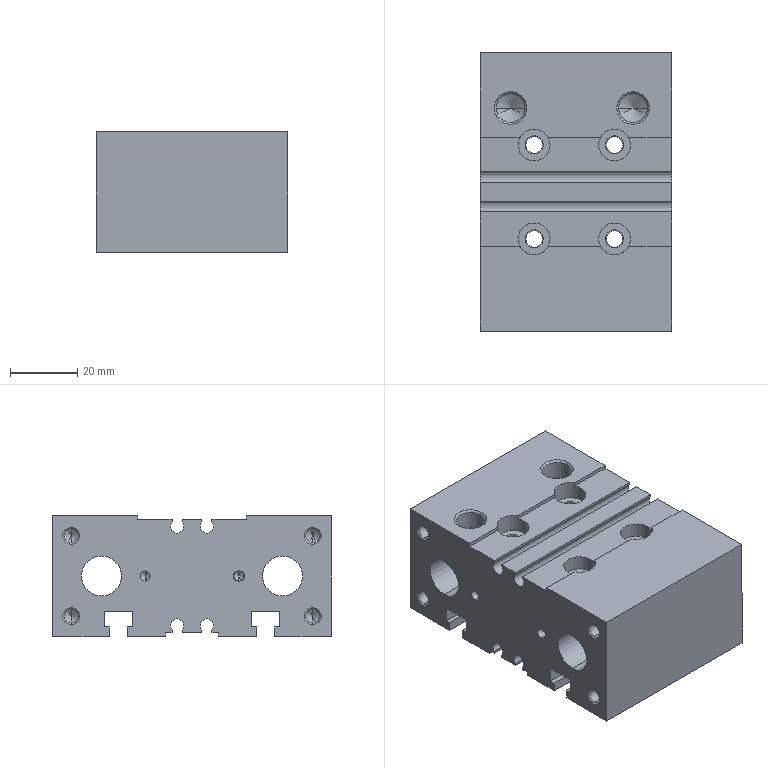Component | SolidWorks | MGPM20-20Z-M9P-1_MGPM20_20Z_0_BODY_2-1 | 1 solid | 176 faces | volume 129991 mm3 | cylinder 64 | plane 64 | cone 48 | commonest cylinder face diameters 3 x12 4.134 x8 9.5 x8 5.4 x8 4.917 x8 8.566 x8 4.05 x4 12 x4